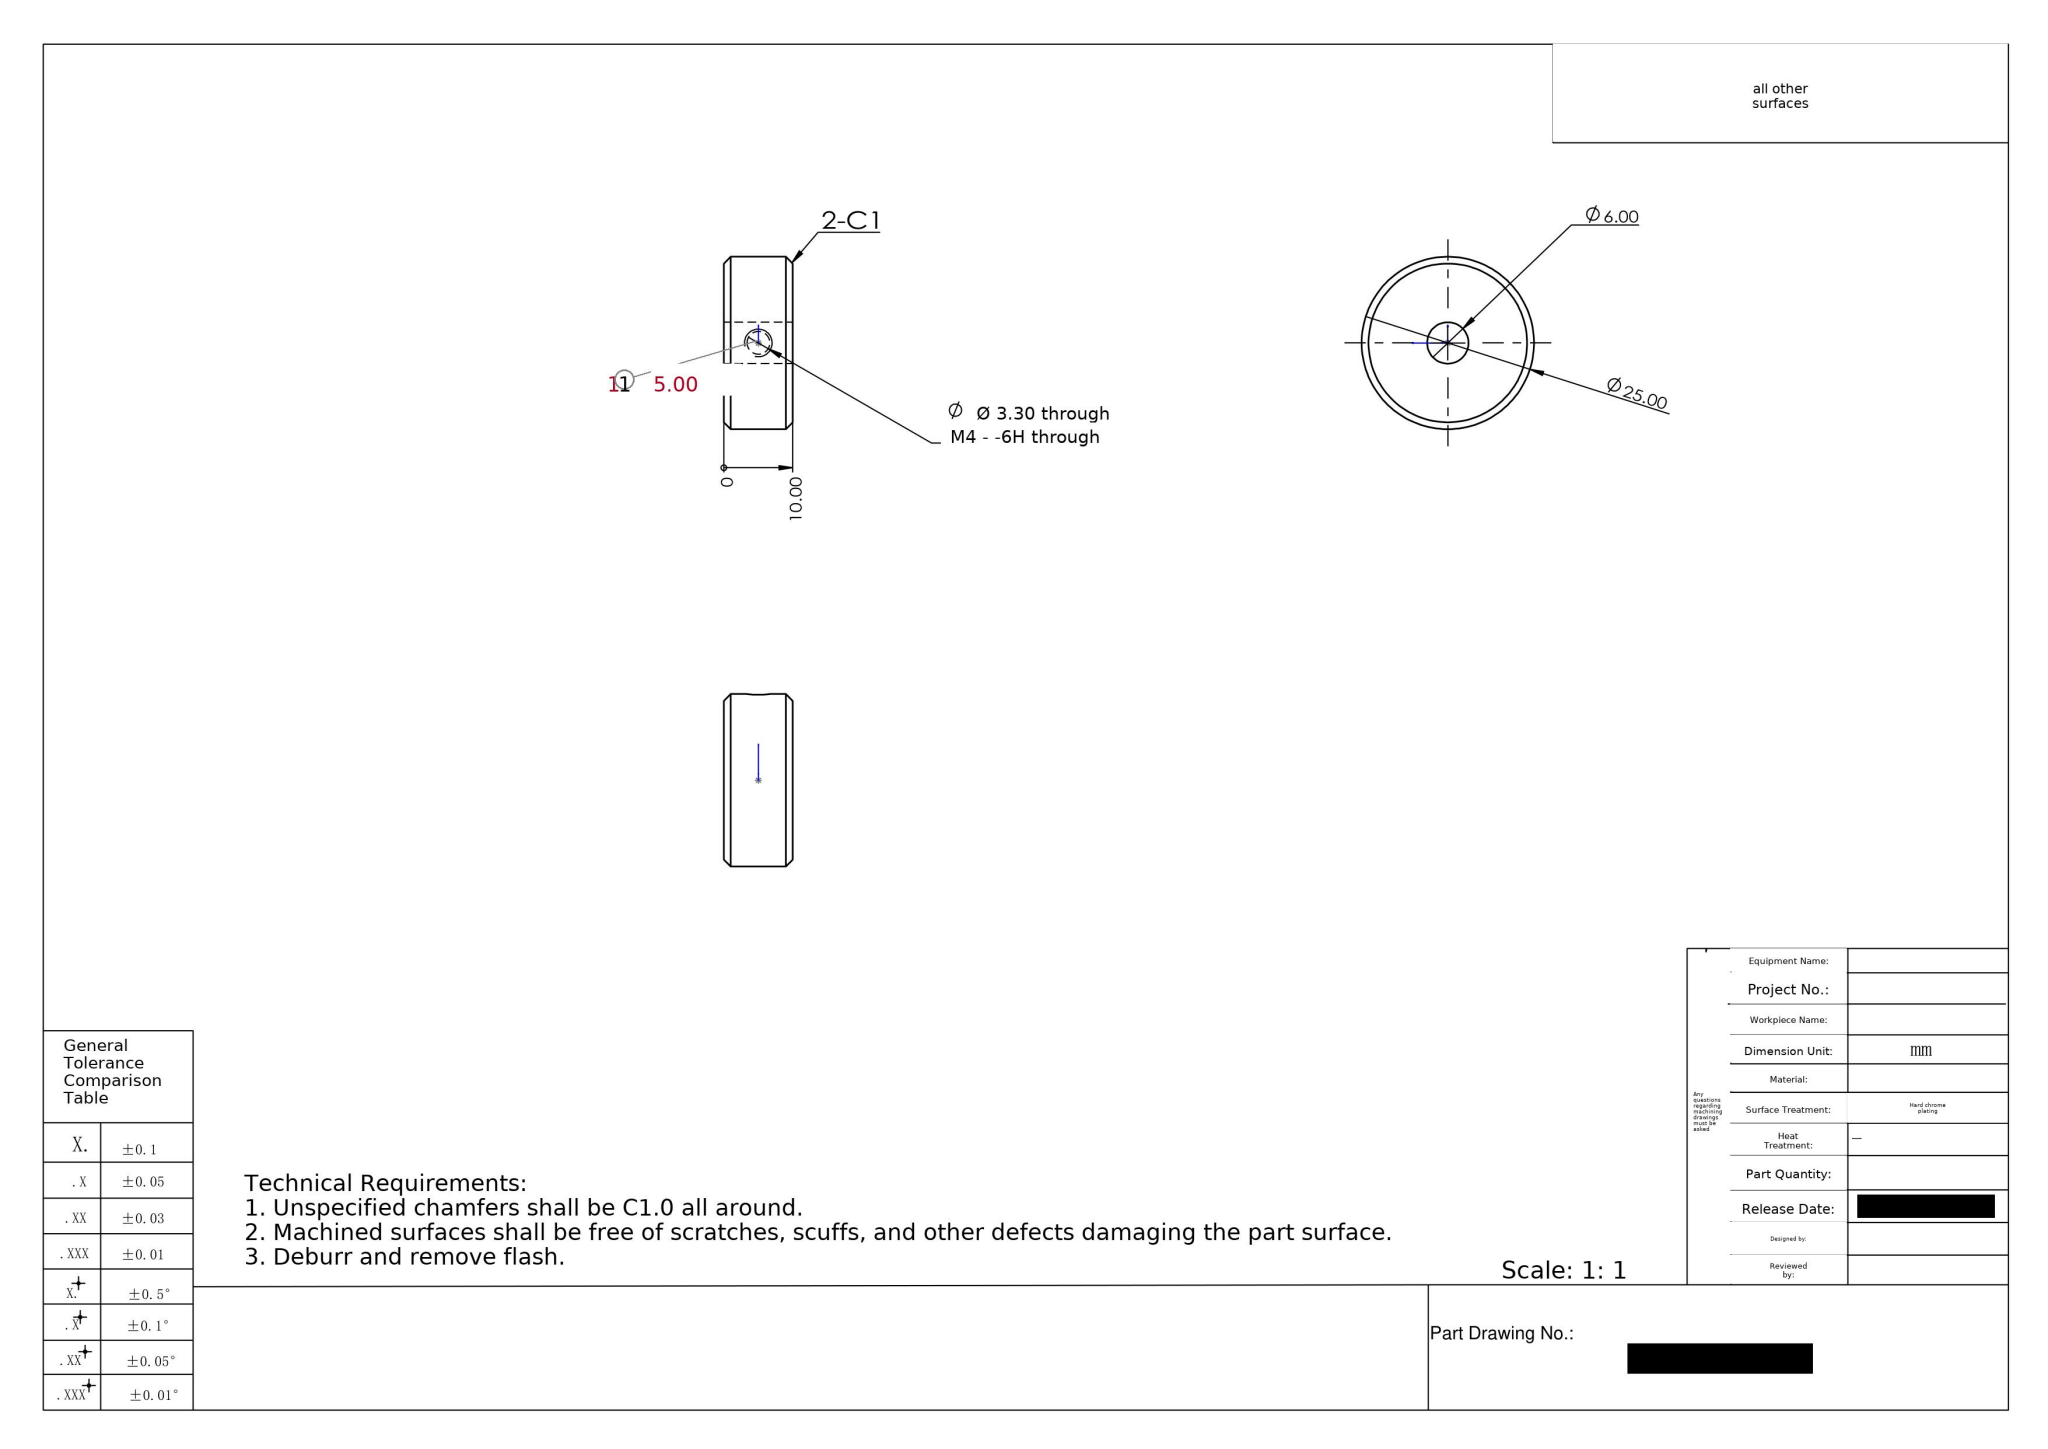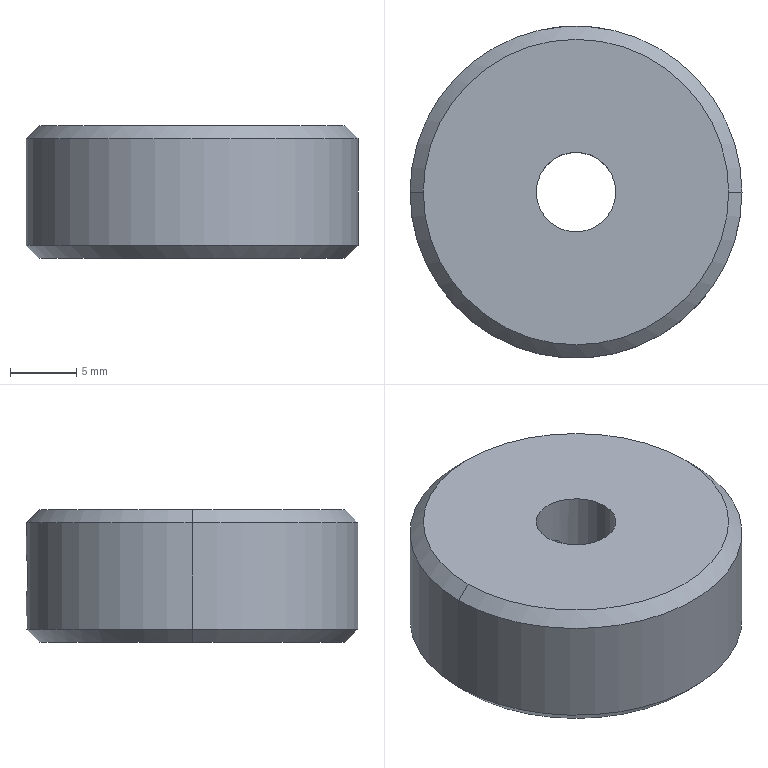Part | SolidWorks | mm | 1 solid | 12 faces | box 25 x 25 x 10 mm | volume 4468 mm3 | cylinder 6 | cone 4 | plane 2 | commonest cylinder face diameters 3.3 x2 6 x2 25 x2
build123d program:
from build123d import *

# Parameters (mm, degrees)
SKETCH1_R              = 12.5
SKETCH1_R_2            = 3
EXTRUDE1_DEPTH         = 5
M4_TAPPED_HOLE1_REACH  = 30.395
M4_TAPPED_HOLE1_BORE_R = 1.65
CHAMFER1_SIZE          = 1


with BuildPart() as part:
    # Sketch1 → Extrude1 (new, symmetric)
    with BuildSketch(Plane.XY):
        Circle(SKETCH1_R)
        Circle(SKETCH1_R_2, mode=Mode.SUBTRACT)
    extrude(amount=EXTRUDE1_DEPTH, both=True)

    # M4 Tapped Hole1 bore (on position points) → M4 Tapped Hole1 (cut, up to next)
    with BuildSketch(Plane(origin=(0, 12.5, 0), x_dir=(1, 0, 0), z_dir=(0, 1, 0)), mode=Mode.PRIVATE) as m4_tapped_hole1_sk1:
        Circle(M4_TAPPED_HOLE1_BORE_R)
    m4_tapped_hole1_tool1 = extrude(m4_tapped_hole1_sk1.sketch, amount=-M4_TAPPED_HOLE1_REACH, mode=Mode.PRIVATE) & part.part
    add(m4_tapped_hole1_tool1.solids().sort_by_distance((0, 12.5, 0))[0], mode=Mode.SUBTRACT)

    # Chamfer1
    chamfer1_edges = [part.edges().sort_by_distance(p)[0] for p in [
        (-12.5, 0, -5),
        (-12.5, 0, 5),
    ]]
    chamfer(chamfer1_edges, length=CHAMFER1_SIZE)


solid = part.part
STEP:
#1=CARTESIAN_POINT('',(-11.5,0.,-5.));
#2=VERTEX_POINT('',#1);
#3=CARTESIAN_POINT('',(11.5,0.,-5.));
#4=VERTEX_POINT('',#3);
#5=CARTESIAN_POINT('',(0.,0.,-5.));
#6=DIRECTION('',(0.,0.,-1.));
#7=DIRECTION('',(1.,0.,0.));
#8=AXIS2_PLACEMENT_3D('',#5,#6,#7);
#9=CIRCLE('',#8,11.5);
#10=EDGE_CURVE('',#2,#4,#9,.T.);
#11=ORIENTED_EDGE('',*,*,#10,.F.);
#12=CARTESIAN_POINT('',(-12.5,0.,-4.));
#13=VERTEX_POINT('',#12);
#14=CARTESIAN_POINT('',(-12.5,0.,-4.));
#15=DIRECTION('',(-0.7071,0.,0.7071));
#16=VECTOR('',#15,1000.);
#17=LINE('',#14,#16);
#18=EDGE_CURVE('',#2,#13,#17,.T.);
#19=ORIENTED_EDGE('',*,*,#18,.T.);
#20=CARTESIAN_POINT('',(12.5,0.,-4.));
#21=VERTEX_POINT('',#20);
#22=CARTESIAN_POINT('',(0.,0.,-4.));
#23=DIRECTION('',(0.,0.,1.));
#24=DIRECTION('',(1.,0.,0.));
#25=AXIS2_PLACEMENT_3D('',#22,#23,#24);
#26=CIRCLE('',#25,12.5);
#27=EDGE_CURVE('',#21,#13,#26,.T.);
#28=ORIENTED_EDGE('',*,*,#27,.F.);
#29=CARTESIAN_POINT('',(12.5,0.,-4.));
#30=DIRECTION('',(0.7071,0.,0.7071));
#31=VECTOR('',#30,1000.);
#32=LINE('',#29,#31);
#33=EDGE_CURVE('',#4,#21,#32,.T.);
#34=ORIENTED_EDGE('',*,*,#33,.F.);
#35=EDGE_LOOP('',(#11,#19,#28,#34));
#36=FACE_OUTER_BOUND('',#35,.T.);
#37=CARTESIAN_POINT('',(0.,0.,-4.));
#38=DIRECTION('',(0.,0.,1.));
#39=DIRECTION('',(1.,0.,0.));
#40=AXIS2_PLACEMENT_3D('',#37,#38,#39);
#41=CONICAL_SURFACE('',#40,12.5,0.7854);
#42=ADVANCED_FACE('',(#36),#41,.T.);
#43=CARTESIAN_POINT('',(11.5,0.,5.));
#44=VERTEX_POINT('',#43);
#45=CARTESIAN_POINT('',(-11.5,0.,5.));
#46=VERTEX_POINT('',#45);
#47=CARTESIAN_POINT('',(0.,0.,5.));
#48=DIRECTION('',(0.,0.,1.));
#49=DIRECTION('',(1.,0.,0.));
#50=AXIS2_PLACEMENT_3D('',#47,#48,#49);
#51=CIRCLE('',#50,11.5);
#52=EDGE_CURVE('',#44,#46,#51,.T.);
#53=ORIENTED_EDGE('',*,*,#52,.F.);
#54=CARTESIAN_POINT('',(12.5,0.,4.));
#55=VERTEX_POINT('',#54);
#56=CARTESIAN_POINT('',(11.5,0.,5.));
#57=DIRECTION('',(0.7071,0.,-0.7071));
#58=VECTOR('',#57,1000.);
#59=LINE('',#56,#58);
#60=EDGE_CURVE('',#44,#55,#59,.T.);
#61=ORIENTED_EDGE('',*,*,#60,.T.);
#62=CARTESIAN_POINT('',(-12.5,0.,4.));
#63=VERTEX_POINT('',#62);
#64=CARTESIAN_POINT('',(0.,0.,4.));
#65=DIRECTION('',(0.,0.,-1.));
#66=DIRECTION('',(1.,0.,0.));
#67=AXIS2_PLACEMENT_3D('',#64,#65,#66);
#68=CIRCLE('',#67,12.5);
#69=EDGE_CURVE('',#63,#55,#68,.T.);
#70=ORIENTED_EDGE('',*,*,#69,.F.);
#71=CARTESIAN_POINT('',(-11.5,0.,5.));
#72=DIRECTION('',(-0.7071,0.,-0.7071));
#73=VECTOR('',#72,1000.);
#74=LINE('',#71,#73);
#75=EDGE_CURVE('',#46,#63,#74,.T.);
#76=ORIENTED_EDGE('',*,*,#75,.F.);
#77=EDGE_LOOP('',(#53,#61,#70,#76));
#78=FACE_OUTER_BOUND('',#77,.T.);
#79=CARTESIAN_POINT('',(0.,0.,5.));
#80=DIRECTION('',(0.,0.,-1.));
#81=DIRECTION('',(-1.,0.,0.));
#82=AXIS2_PLACEMENT_3D('',#79,#80,#81);
#83=CONICAL_SURFACE('',#82,11.5,0.7854);
#84=ADVANCED_FACE('',(#78),#83,.T.);
#85=CARTESIAN_POINT('',(-0.,3.,1.65));
#86=VERTEX_POINT('',#85);
#87=CARTESIAN_POINT('',(0.,3.,-1.65));
#88=VERTEX_POINT('',#87);
#89=CARTESIAN_POINT('',(-0.,3.,1.65));
#90=CARTESIAN_POINT('',(-0.1115,3.,1.65));
#91=CARTESIAN_POINT('',(-0.2208,2.994,1.639));
#92=CARTESIAN_POINT('',(-0.435,2.97,1.595));
#93=CARTESIAN_POINT('',(-0.541,2.953,1.563));
#94=CARTESIAN_POINT('',(-0.8399,2.887,1.437));
#95=CARTESIAN_POINT('',(-1.02,2.826,1.314));
#96=CARTESIAN_POINT('',(-1.317,2.7,1.016));
#97=CARTESIAN_POINT('',(-1.438,2.635,0.8367));
#98=CARTESIAN_POINT('',(-1.563,2.561,0.5406));
#99=CARTESIAN_POINT('',(-1.595,2.541,0.4349));
#100=CARTESIAN_POINT('',(-1.639,2.513,0.2211));
#101=CARTESIAN_POINT('',(-1.65,2.506,0.1125));
#102=CARTESIAN_POINT('',(-1.65,2.505,-0.1082));
#103=CARTESIAN_POINT('',(-1.639,2.513,-0.2198));
#104=CARTESIAN_POINT('',(-1.596,2.541,-0.434));
#105=CARTESIAN_POINT('',(-1.563,2.561,-0.5391));
#106=CARTESIAN_POINT('',(-1.438,2.635,-0.8379));
#107=CARTESIAN_POINT('',(-1.316,2.701,-1.017));
#108=CARTESIAN_POINT('',(-1.018,2.826,-1.315));
#109=CARTESIAN_POINT('',(-0.838,2.888,-1.438));
#110=CARTESIAN_POINT('',(-0.5406,2.953,-1.563));
#111=CARTESIAN_POINT('',(-0.4348,2.97,-1.595));
#112=CARTESIAN_POINT('',(-0.2193,2.994,-1.639));
#113=CARTESIAN_POINT('',(-0.1103,3.,-1.65));
#114=CARTESIAN_POINT('',(0.,3.,-1.65));
#115=B_SPLINE_CURVE_WITH_KNOTS('',3,(#89,#90,#91,#92,#93,#94,#95,#96,#97,#98,#99,#100,#101,#102,#103,#104,#105,#106,#107,#108,#109,#110,#111,#112,#113,#114),.UNSPECIFIED.,.F.,.F.,(4,2,2,2,2,2,2,2,2,2,2,2,4),(0.,0.0003294,0.0006588,0.001318,0.001976,0.002306,0.002635,0.002965,0.003294,0.003953,0.004612,0.004941,0.00527),.UNSPECIFIED.);
#116=EDGE_CURVE('',#86,#88,#115,.T.);
#117=ORIENTED_EDGE('',*,*,#116,.T.);
#118=CARTESIAN_POINT('',(0.,12.5,-1.65));
#119=VERTEX_POINT('',#118);
#120=CARTESIAN_POINT('',(0.,12.5,-1.65));
#121=DIRECTION('',(0.,1.,0.));
#122=VECTOR('',#121,1000.);
#123=LINE('',#120,#122);
#124=EDGE_CURVE('',#88,#119,#123,.T.);
#125=ORIENTED_EDGE('',*,*,#124,.T.);
#126=CARTESIAN_POINT('',(-0.,12.5,1.65));
#127=VERTEX_POINT('',#126);
#128=CARTESIAN_POINT('',(-0.,12.5,1.65));
#129=CARTESIAN_POINT('',(-0.1091,12.5,1.65));
#130=CARTESIAN_POINT('',(-0.2164,12.499,1.639));
#131=CARTESIAN_POINT('',(-0.4275,12.493,1.597));
#132=CARTESIAN_POINT('',(-0.5324,12.489,1.565));
#133=CARTESIAN_POINT('',(-0.7322,12.479,1.483));
#134=CARTESIAN_POINT('',(-0.8269,12.473,1.432));
#135=CARTESIAN_POINT('',(-1.006,12.46,1.312));
#136=CARTESIAN_POINT('',(-1.091,12.453,1.243));
#137=CARTESIAN_POINT('',(-1.319,12.431,1.014));
#138=CARTESIAN_POINT('',(-1.442,12.417,0.8305));
#139=CARTESIAN_POINT('',(-1.606,12.397,0.4334));
#140=CARTESIAN_POINT('',(-1.65,12.391,0.2161));
#141=CARTESIAN_POINT('',(-1.65,12.391,-0.1071));
#142=CARTESIAN_POINT('',(-1.639,12.392,-0.2166));
#143=CARTESIAN_POINT('',(-1.597,12.398,-0.4283));
#144=CARTESIAN_POINT('',(-1.566,12.402,-0.5312));
#145=CARTESIAN_POINT('',(-1.483,12.412,-0.7312));
#146=CARTESIAN_POINT('',(-1.431,12.418,-0.8276));
#147=CARTESIAN_POINT('',(-1.312,12.431,-1.006));
#148=CARTESIAN_POINT('',(-1.244,12.438,-1.09));
#149=CARTESIAN_POINT('',(-1.09,12.453,-1.244));
#150=CARTESIAN_POINT('',(-1.007,12.46,-1.312));
#151=CARTESIAN_POINT('',(-0.8281,12.473,-1.431));
#152=CARTESIAN_POINT('',(-0.7315,12.479,-1.483));
#153=CARTESIAN_POINT('',(-0.5318,12.489,-1.566));
#154=CARTESIAN_POINT('',(-0.4289,12.493,-1.597));
#155=CARTESIAN_POINT('',(-0.2172,12.499,-1.639));
#156=CARTESIAN_POINT('',(-0.1077,12.5,-1.65));
#157=CARTESIAN_POINT('',(0.,12.5,-1.65));
#158=B_SPLINE_CURVE_WITH_KNOTS('',3,(#128,#129,#130,#131,#132,#133,#134,#135,#136,#137,#138,#139,#140,#141,#142,#143,#144,#145,#146,#147,#148,#149,#150,#151,#152,#153,#154,#155,#156,#157),.UNSPECIFIED.,.F.,.F.,(4,2,2,2,2,2,2,2,2,2,2,2,2,2,4),(0.,0.0003228,0.0006455,0.0009683,0.001291,0.001937,0.002582,0.002905,0.003228,0.00355,0.003873,0.004196,0.004519,0.004842,0.005164),.UNSPECIFIED.);
#159=EDGE_CURVE('',#127,#119,#158,.T.);
#160=ORIENTED_EDGE('',*,*,#159,.F.);
#161=CARTESIAN_POINT('',(0.,12.5,1.65));
#162=DIRECTION('',(0.,1.,0.));
#163=VECTOR('',#162,1000.);
#164=LINE('',#161,#163);
#165=EDGE_CURVE('',#86,#127,#164,.T.);
#166=ORIENTED_EDGE('',*,*,#165,.F.);
#167=EDGE_LOOP('',(#117,#125,#160,#166));
#168=FACE_OUTER_BOUND('',#167,.T.);
#169=CARTESIAN_POINT('',(0.,12.5,0.));
#170=DIRECTION('',(0.,1.,0.));
#171=DIRECTION('',(0.,0.,1.));
#172=AXIS2_PLACEMENT_3D('',#169,#170,#171);
#173=CYLINDRICAL_SURFACE('',#172,1.65);
#174=ADVANCED_FACE('',(#168),#173,.F.);
#175=CARTESIAN_POINT('',(-3.,0.,5.));
#176=VERTEX_POINT('',#175);
#177=CARTESIAN_POINT('',(3.,0.,5.));
#178=VERTEX_POINT('',#177);
#179=CARTESIAN_POINT('',(0.,0.,5.));
#180=DIRECTION('',(0.,0.,1.));
#181=DIRECTION('',(1.,0.,0.));
#182=AXIS2_PLACEMENT_3D('',#179,#180,#181);
#183=CIRCLE('',#182,3.);
#184=EDGE_CURVE('',#176,#178,#183,.T.);
#185=ORIENTED_EDGE('',*,*,#184,.T.);
#186=CARTESIAN_POINT('',(3.,0.,-5.));
#187=VERTEX_POINT('',#186);
#188=CARTESIAN_POINT('',(3.,0.,5.));
#189=DIRECTION('',(0.,0.,-1.));
#190=VECTOR('',#189,1000.);
#191=LINE('',#188,#190);
#192=EDGE_CURVE('',#178,#187,#191,.T.);
#193=ORIENTED_EDGE('',*,*,#192,.T.);
#194=CARTESIAN_POINT('',(-3.,0.,-5.));
#195=VERTEX_POINT('',#194);
#196=CARTESIAN_POINT('',(0.,0.,-5.));
#197=DIRECTION('',(0.,0.,1.));
#198=DIRECTION('',(1.,0.,0.));
#199=AXIS2_PLACEMENT_3D('',#196,#197,#198);
#200=CIRCLE('',#199,3.);
#201=EDGE_CURVE('',#195,#187,#200,.T.);
#202=ORIENTED_EDGE('',*,*,#201,.F.);
#203=CARTESIAN_POINT('',(-3.,0.,5.));
#204=DIRECTION('',(0.,0.,-1.));
#205=VECTOR('',#204,1000.);
#206=LINE('',#203,#205);
#207=EDGE_CURVE('',#176,#195,#206,.T.);
#208=ORIENTED_EDGE('',*,*,#207,.F.);
#209=EDGE_LOOP('',(#185,#193,#202,#208));
#210=FACE_OUTER_BOUND('',#209,.T.);
#211=CARTESIAN_POINT('',(0.,0.,5.));
#212=DIRECTION('',(0.,0.,-1.));
#213=DIRECTION('',(-1.,0.,0.));
#214=AXIS2_PLACEMENT_3D('',#211,#212,#213);
#215=CYLINDRICAL_SURFACE('',#214,3.);
#216=ADVANCED_FACE('',(#210),#215,.F.);
#217=ORIENTED_EDGE('',*,*,#159,.T.);
#218=CARTESIAN_POINT('',(0.,12.5,-1.65));
#219=CARTESIAN_POINT('',(0.2154,12.5,-1.65));
#220=CARTESIAN_POINT('',(0.4327,12.494,-1.607));
#221=CARTESIAN_POINT('',(0.8299,12.474,-1.442));
#222=CARTESIAN_POINT('',(1.014,12.46,-1.319));
#223=CARTESIAN_POINT('',(1.242,12.438,-1.092));
#224=CARTESIAN_POINT('',(1.312,12.431,-1.007));
#225=CARTESIAN_POINT('',(1.431,12.418,-0.8277));
#226=CARTESIAN_POINT('',(1.482,12.412,-0.733));
#227=CARTESIAN_POINT('',(1.565,12.402,-0.5333));
#228=CARTESIAN_POINT('',(1.597,12.398,-0.4285));
#229=CARTESIAN_POINT('',(1.639,12.392,-0.2176));
#230=CARTESIAN_POINT('',(1.65,12.391,-0.1102));
#231=CARTESIAN_POINT('',(1.65,12.391,0.1079));
#232=CARTESIAN_POINT('',(1.639,12.392,0.2152));
#233=CARTESIAN_POINT('',(1.598,12.398,0.4263));
#234=CARTESIAN_POINT('',(1.566,12.402,0.5312));
#235=CARTESIAN_POINT('',(1.483,12.412,0.7309));
#236=CARTESIAN_POINT('',(1.433,12.418,0.8257));
#237=CARTESIAN_POINT('',(1.313,12.431,1.005));
#238=CARTESIAN_POINT('',(1.243,12.438,1.09));
#239=CARTESIAN_POINT('',(1.016,12.46,1.318));
#240=CARTESIAN_POINT('',(0.8319,12.474,1.441));
#241=CARTESIAN_POINT('',(0.4351,12.494,1.606));
#242=CARTESIAN_POINT('',(0.2182,12.5,1.65));
#243=CARTESIAN_POINT('',(-0.,12.5,1.65));
#244=B_SPLINE_CURVE_WITH_KNOTS('',3,(#218,#219,#220,#221,#222,#223,#224,#225,#226,#227,#228,#229,#230,#231,#232,#233,#234,#235,#236,#237,#238,#239,#240,#241,#242,#243),.UNSPECIFIED.,.F.,.F.,(4,2,2,2,2,2,2,2,2,2,2,2,4),(0.005164,0.00581,0.006455,0.006778,0.0071,0.007423,0.007746,0.008068,0.008391,0.008714,0.009037,0.009682,0.01033),.UNSPECIFIED.);
#245=EDGE_CURVE('',#119,#127,#244,.T.);
#246=ORIENTED_EDGE('',*,*,#245,.T.);
#247=EDGE_LOOP('',(#217,#246));
#248=FACE_BOUND('',#247,.T.);
#249=ORIENTED_EDGE('',*,*,#69,.T.);
#250=CARTESIAN_POINT('',(12.5,0.,5.));
#251=DIRECTION('',(0.,0.,-1.));
#252=VECTOR('',#251,1000.);
#253=LINE('',#250,#252);
#254=EDGE_CURVE('',#55,#21,#253,.T.);
#255=ORIENTED_EDGE('',*,*,#254,.T.);
#256=ORIENTED_EDGE('',*,*,#27,.T.);
#257=CARTESIAN_POINT('',(-12.5,0.,5.));
#258=DIRECTION('',(0.,0.,-1.));
#259=VECTOR('',#258,1000.);
#260=LINE('',#257,#259);
#261=EDGE_CURVE('',#63,#13,#260,.T.);
#262=ORIENTED_EDGE('',*,*,#261,.F.);
#263=EDGE_LOOP('',(#249,#255,#256,#262));
#264=FACE_OUTER_BOUND('',#263,.T.);
#265=CARTESIAN_POINT('',(0.,0.,5.));
#266=DIRECTION('',(0.,0.,-1.));
#267=DIRECTION('',(-1.,0.,0.));
#268=AXIS2_PLACEMENT_3D('',#265,#266,#267);
#269=CYLINDRICAL_SURFACE('',#268,12.5);
#270=ADVANCED_FACE('',(#248,#264),#269,.T.);
#271=CARTESIAN_POINT('',(0.,0.,5.));
#272=DIRECTION('',(0.,0.,1.));
#273=DIRECTION('',(1.,0.,0.));
#274=AXIS2_PLACEMENT_3D('',#271,#272,#273);
#275=CIRCLE('',#274,11.5);
#276=EDGE_CURVE('',#46,#44,#275,.T.);
#277=ORIENTED_EDGE('',*,*,#276,.T.);
#278=ORIENTED_EDGE('',*,*,#52,.T.);
#279=EDGE_LOOP('',(#277,#278));
#280=FACE_OUTER_BOUND('',#279,.T.);
#281=ORIENTED_EDGE('',*,*,#184,.F.);
#282=CARTESIAN_POINT('',(0.,0.,5.));
#283=DIRECTION('',(0.,0.,1.));
#284=DIRECTION('',(1.,0.,0.));
#285=AXIS2_PLACEMENT_3D('',#282,#283,#284);
#286=CIRCLE('',#285,3.);
#287=EDGE_CURVE('',#178,#176,#286,.T.);
#288=ORIENTED_EDGE('',*,*,#287,.F.);
#289=EDGE_LOOP('',(#281,#288));
#290=FACE_BOUND('',#289,.T.);
#291=CARTESIAN_POINT('',(0.,0.,5.));
#292=DIRECTION('',(0.,0.,1.));
#293=DIRECTION('',(1.,0.,0.));
#294=AXIS2_PLACEMENT_3D('',#291,#292,#293);
#295=PLANE('',#294);
#296=ADVANCED_FACE('',(#280,#290),#295,.T.);
#297=CARTESIAN_POINT('',(0.,0.,-5.));
#298=DIRECTION('',(0.,0.,-1.));
#299=DIRECTION('',(1.,0.,0.));
#300=AXIS2_PLACEMENT_3D('',#297,#298,#299);
#301=CIRCLE('',#300,11.5);
#302=EDGE_CURVE('',#4,#2,#301,.T.);
#303=ORIENTED_EDGE('',*,*,#302,.T.);
#304=ORIENTED_EDGE('',*,*,#10,.T.);
#305=EDGE_LOOP('',(#303,#304));
#306=FACE_OUTER_BOUND('',#305,.T.);
#307=ORIENTED_EDGE('',*,*,#201,.T.);
#308=CARTESIAN_POINT('',(0.,0.,-5.));
#309=DIRECTION('',(0.,0.,1.));
#310=DIRECTION('',(1.,0.,0.));
#311=AXIS2_PLACEMENT_3D('',#308,#309,#310);
#312=CIRCLE('',#311,3.);
#313=EDGE_CURVE('',#187,#195,#312,.T.);
#314=ORIENTED_EDGE('',*,*,#313,.T.);
#315=EDGE_LOOP('',(#307,#314));
#316=FACE_BOUND('',#315,.T.);
#317=CARTESIAN_POINT('',(0.,0.,-5.));
#318=DIRECTION('',(0.,0.,1.));
#319=DIRECTION('',(1.,0.,0.));
#320=AXIS2_PLACEMENT_3D('',#317,#318,#319);
#321=PLANE('',#320);
#322=ADVANCED_FACE('',(#306,#316),#321,.F.);
#323=ORIENTED_EDGE('',*,*,#254,.F.);
#324=CARTESIAN_POINT('',(0.,0.,4.));
#325=DIRECTION('',(0.,0.,-1.));
#326=DIRECTION('',(1.,0.,0.));
#327=AXIS2_PLACEMENT_3D('',#324,#325,#326);
#328=CIRCLE('',#327,12.5);
#329=EDGE_CURVE('',#55,#63,#328,.T.);
#330=ORIENTED_EDGE('',*,*,#329,.T.);
#331=ORIENTED_EDGE('',*,*,#261,.T.);
#332=CARTESIAN_POINT('',(0.,0.,-4.));
#333=DIRECTION('',(0.,0.,1.));
#334=DIRECTION('',(1.,0.,0.));
#335=AXIS2_PLACEMENT_3D('',#332,#333,#334);
#336=CIRCLE('',#335,12.5);
#337=EDGE_CURVE('',#13,#21,#336,.T.);
#338=ORIENTED_EDGE('',*,*,#337,.T.);
#339=EDGE_LOOP('',(#323,#330,#331,#338));
#340=FACE_OUTER_BOUND('',#339,.T.);
#341=CARTESIAN_POINT('',(0.,0.,5.));
#342=DIRECTION('',(0.,0.,-1.));
#343=DIRECTION('',(-1.,0.,0.));
#344=AXIS2_PLACEMENT_3D('',#341,#342,#343);
#345=CYLINDRICAL_SURFACE('',#344,12.5);
#346=ADVANCED_FACE('',(#340),#345,.T.);
#347=ORIENTED_EDGE('',*,*,#192,.F.);
#348=ORIENTED_EDGE('',*,*,#287,.T.);
#349=ORIENTED_EDGE('',*,*,#207,.T.);
#350=ORIENTED_EDGE('',*,*,#313,.F.);
#351=EDGE_LOOP('',(#347,#348,#349,#350));
#352=FACE_OUTER_BOUND('',#351,.T.);
#353=ORIENTED_EDGE('',*,*,#116,.F.);
#354=CARTESIAN_POINT('',(0.,3.,-1.65));
#355=CARTESIAN_POINT('',(0.11,3.,-1.65));
#356=CARTESIAN_POINT('',(0.2217,2.994,-1.639));
#357=CARTESIAN_POINT('',(0.4359,2.97,-1.595));
#358=CARTESIAN_POINT('',(0.5406,2.953,-1.563));
#359=CARTESIAN_POINT('',(0.741,2.909,-1.478));
#360=CARTESIAN_POINT('',(0.835,2.883,-1.427));
#361=CARTESIAN_POINT('',(1.012,2.826,-1.308));
#362=CARTESIAN_POINT('',(1.094,2.794,-1.239));
#363=CARTESIAN_POINT('',(1.318,2.7,-1.015));
#364=CARTESIAN_POINT('',(1.438,2.634,-0.836));
#365=CARTESIAN_POINT('',(1.604,2.537,-0.4427));
#366=CARTESIAN_POINT('',(1.65,2.506,-0.222));
#367=CARTESIAN_POINT('',(1.65,2.505,0.1068));
#368=CARTESIAN_POINT('',(1.639,2.513,0.2187));
#369=CARTESIAN_POINT('',(1.596,2.54,0.4332));
#370=CARTESIAN_POINT('',(1.564,2.561,0.5369));
#371=CARTESIAN_POINT('',(1.48,2.61,0.7373));
#372=CARTESIAN_POINT('',(1.429,2.638,0.831));
#373=CARTESIAN_POINT('',(1.311,2.699,1.007));
#374=CARTESIAN_POINT('',(1.243,2.732,1.09));
#375=CARTESIAN_POINT('',(1.094,2.795,1.24));
#376=CARTESIAN_POINT('',(1.013,2.825,1.307));
#377=CARTESIAN_POINT('',(0.8357,2.883,1.427));
#378=CARTESIAN_POINT('',(0.7403,2.909,1.478));
#379=CARTESIAN_POINT('',(0.4435,2.974,1.604));
#380=CARTESIAN_POINT('',(0.2225,3.,1.65));
#381=CARTESIAN_POINT('',(-0.,3.,1.65));
#382=B_SPLINE_CURVE_WITH_KNOTS('',3,(#354,#355,#356,#357,#358,#359,#360,#361,#362,#363,#364,#365,#366,#367,#368,#369,#370,#371,#372,#373,#374,#375,#376,#377,#378,#379,#380,#381),.UNSPECIFIED.,.F.,.F.,(4,2,2,2,2,2,2,2,2,2,2,2,2,4),(0.00527,0.005599,0.005928,0.006256,0.006585,0.007242,0.007899,0.008228,0.008556,0.008885,0.009213,0.009542,0.009871,0.01053),.UNSPECIFIED.);
#383=EDGE_CURVE('',#88,#86,#382,.T.);
#384=ORIENTED_EDGE('',*,*,#383,.F.);
#385=EDGE_LOOP('',(#353,#384));
#386=FACE_BOUND('',#385,.T.);
#387=CARTESIAN_POINT('',(0.,0.,5.));
#388=DIRECTION('',(0.,0.,-1.));
#389=DIRECTION('',(-1.,0.,0.));
#390=AXIS2_PLACEMENT_3D('',#387,#388,#389);
#391=CYLINDRICAL_SURFACE('',#390,3.);
#392=ADVANCED_FACE('',(#352,#386),#391,.F.);
#393=ORIENTED_EDGE('',*,*,#124,.F.);
#394=ORIENTED_EDGE('',*,*,#383,.T.);
#395=ORIENTED_EDGE('',*,*,#165,.T.);
#396=ORIENTED_EDGE('',*,*,#245,.F.);
#397=EDGE_LOOP('',(#393,#394,#395,#396));
#398=FACE_OUTER_BOUND('',#397,.T.);
#399=CARTESIAN_POINT('',(0.,12.5,0.));
#400=DIRECTION('',(0.,1.,0.));
#401=DIRECTION('',(0.,0.,1.));
#402=AXIS2_PLACEMENT_3D('',#399,#400,#401);
#403=CYLINDRICAL_SURFACE('',#402,1.65);
#404=ADVANCED_FACE('',(#398),#403,.F.);
#405=ORIENTED_EDGE('',*,*,#60,.F.);
#406=ORIENTED_EDGE('',*,*,#276,.F.);
#407=ORIENTED_EDGE('',*,*,#75,.T.);
#408=ORIENTED_EDGE('',*,*,#329,.F.);
#409=EDGE_LOOP('',(#405,#406,#407,#408));
#410=FACE_OUTER_BOUND('',#409,.T.);
#411=CARTESIAN_POINT('',(0.,0.,5.));
#412=DIRECTION('',(0.,0.,-1.));
#413=DIRECTION('',(-1.,0.,0.));
#414=AXIS2_PLACEMENT_3D('',#411,#412,#413);
#415=CONICAL_SURFACE('',#414,11.5,0.7854);
#416=ADVANCED_FACE('',(#410),#415,.T.);
#417=ORIENTED_EDGE('',*,*,#18,.F.);
#418=ORIENTED_EDGE('',*,*,#302,.F.);
#419=ORIENTED_EDGE('',*,*,#33,.T.);
#420=ORIENTED_EDGE('',*,*,#337,.F.);
#421=EDGE_LOOP('',(#417,#418,#419,#420));
#422=FACE_OUTER_BOUND('',#421,.T.);
#423=CARTESIAN_POINT('',(0.,0.,-4.));
#424=DIRECTION('',(0.,0.,1.));
#425=DIRECTION('',(1.,0.,0.));
#426=AXIS2_PLACEMENT_3D('',#423,#424,#425);
#427=CONICAL_SURFACE('',#426,12.5,0.7854);
#428=ADVANCED_FACE('',(#422),#427,.T.);
#429=CLOSED_SHELL('',(#42,#84,#174,#216,#270,#296,#322,#346,#392,#404,#416,#428));
#430=MANIFOLD_SOLID_BREP('',#429);
#431=CARTESIAN_POINT('',(0.,0.,0.));
#432=DIRECTION('',(0.,0.,1.));
#433=DIRECTION('',(1.,0.,0.));
#434=AXIS2_PLACEMENT_3D('',#431,#432,#433);
#435=(LENGTH_UNIT()NAMED_UNIT(*)SI_UNIT(.MILLI.,.METRE.));
#436=UNCERTAINTY_MEASURE_WITH_UNIT(LENGTH_MEASURE(0.00001),#435,'','');
#437=(NAMED_UNIT(*)PLANE_ANGLE_UNIT()SI_UNIT($,.RADIAN.));
#438=(NAMED_UNIT(*)SI_UNIT($,.STERADIAN.)SOLID_ANGLE_UNIT());
#439=(GEOMETRIC_REPRESENTATION_CONTEXT(3)GLOBAL_UNCERTAINTY_ASSIGNED_CONTEXT((#436))GLOBAL_UNIT_ASSIGNED_CONTEXT((#435,#437,#438))REPRESENTATION_CONTEXT('',''));
#440=ADVANCED_BREP_SHAPE_REPRESENTATION('',(#430,#434),#439);